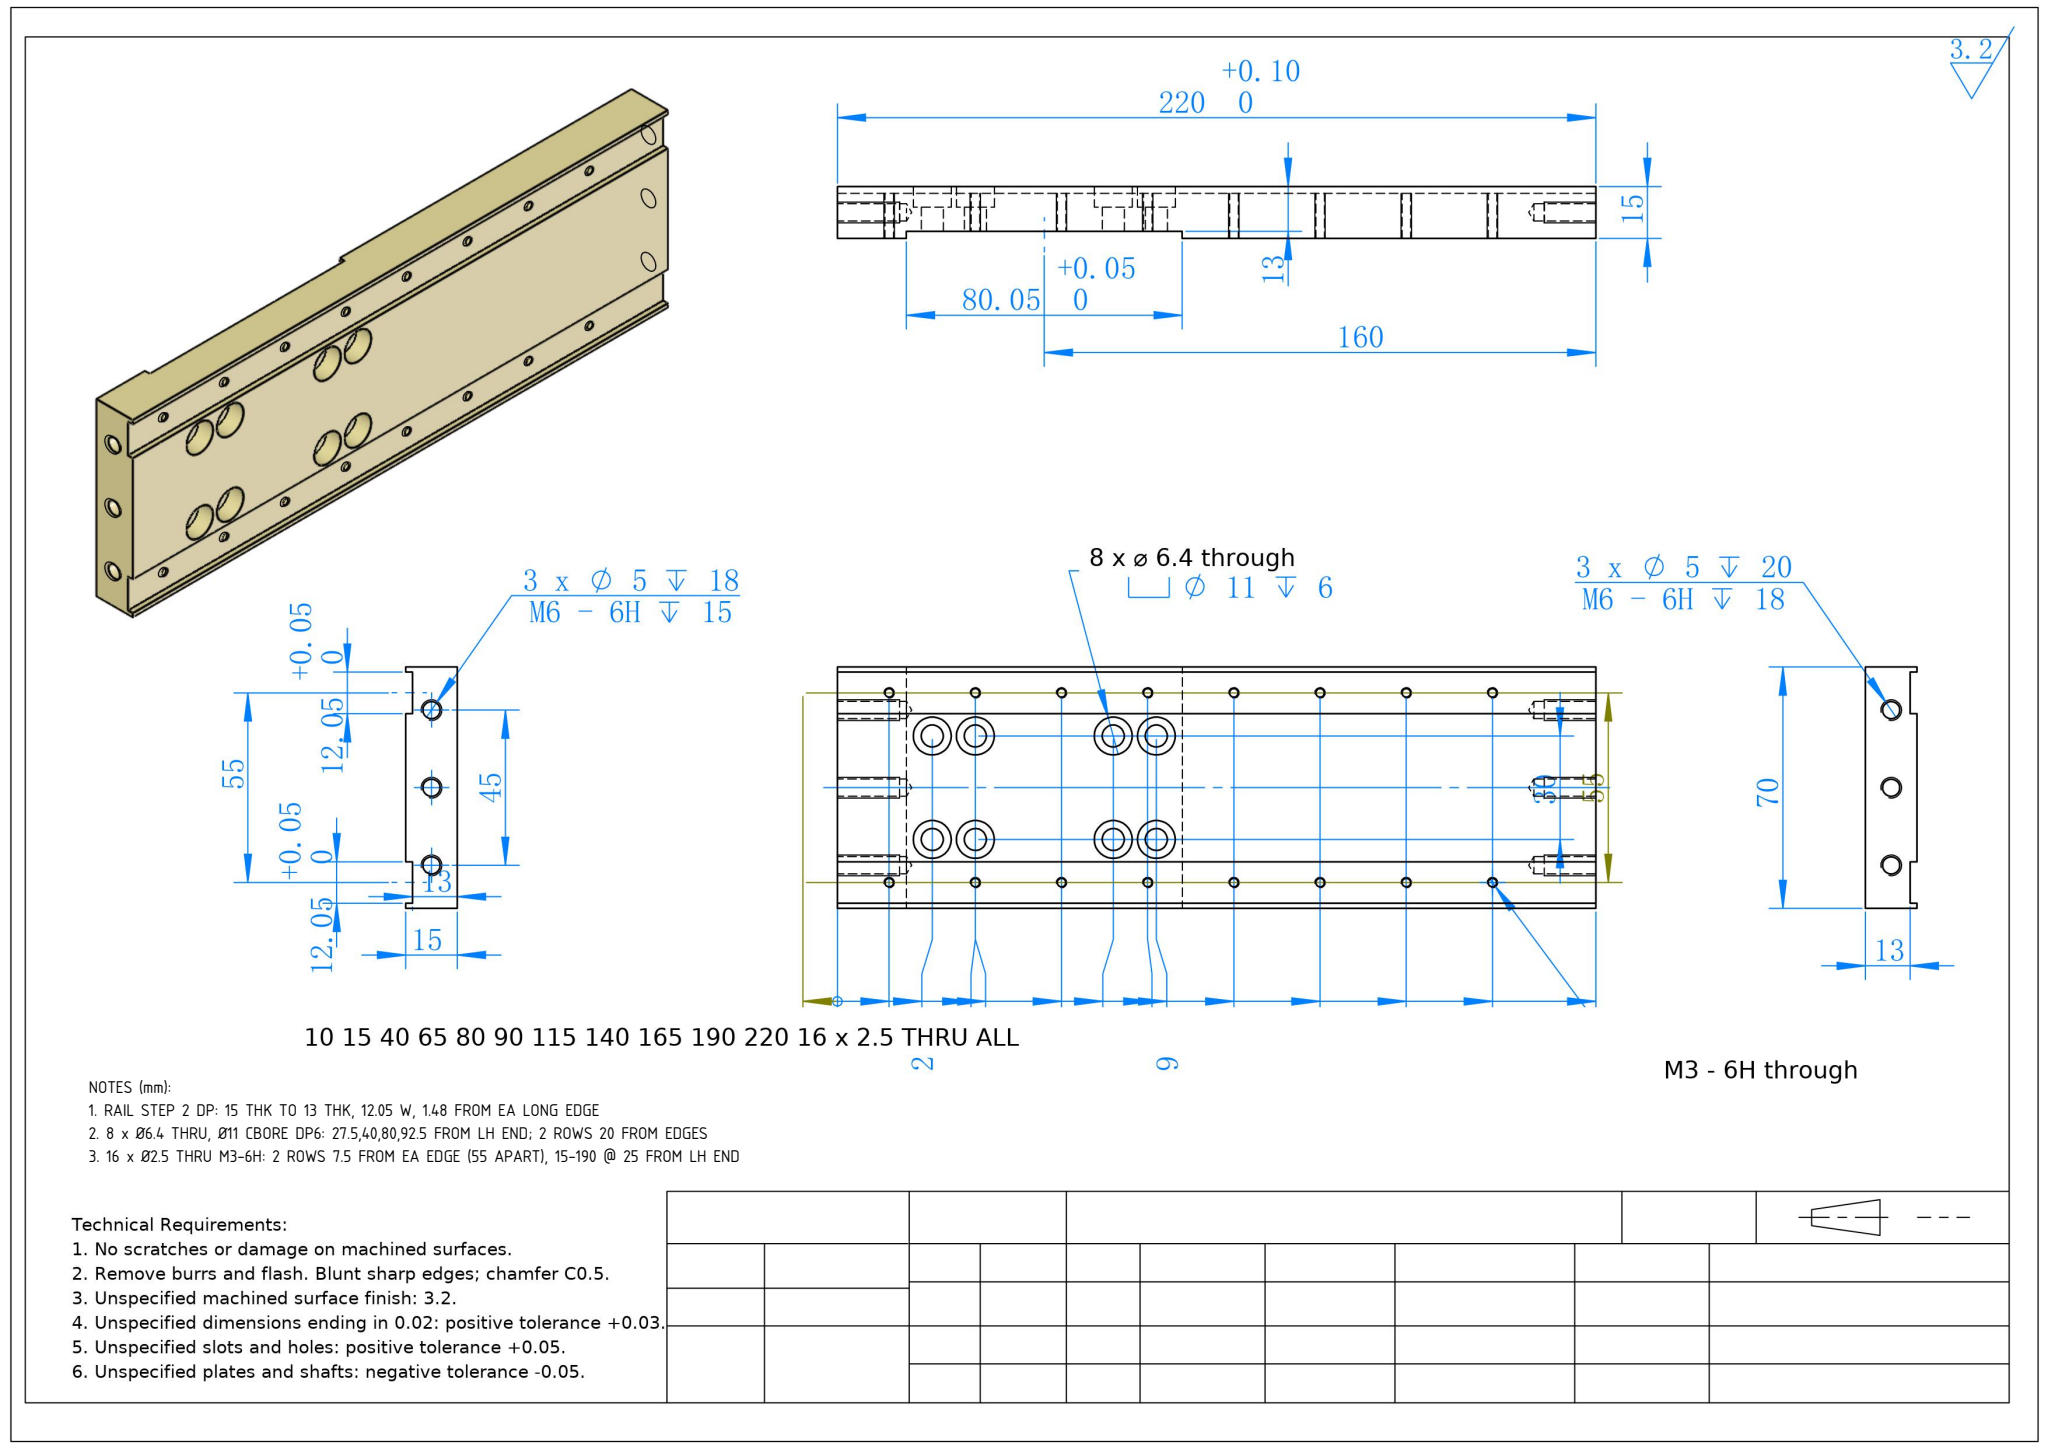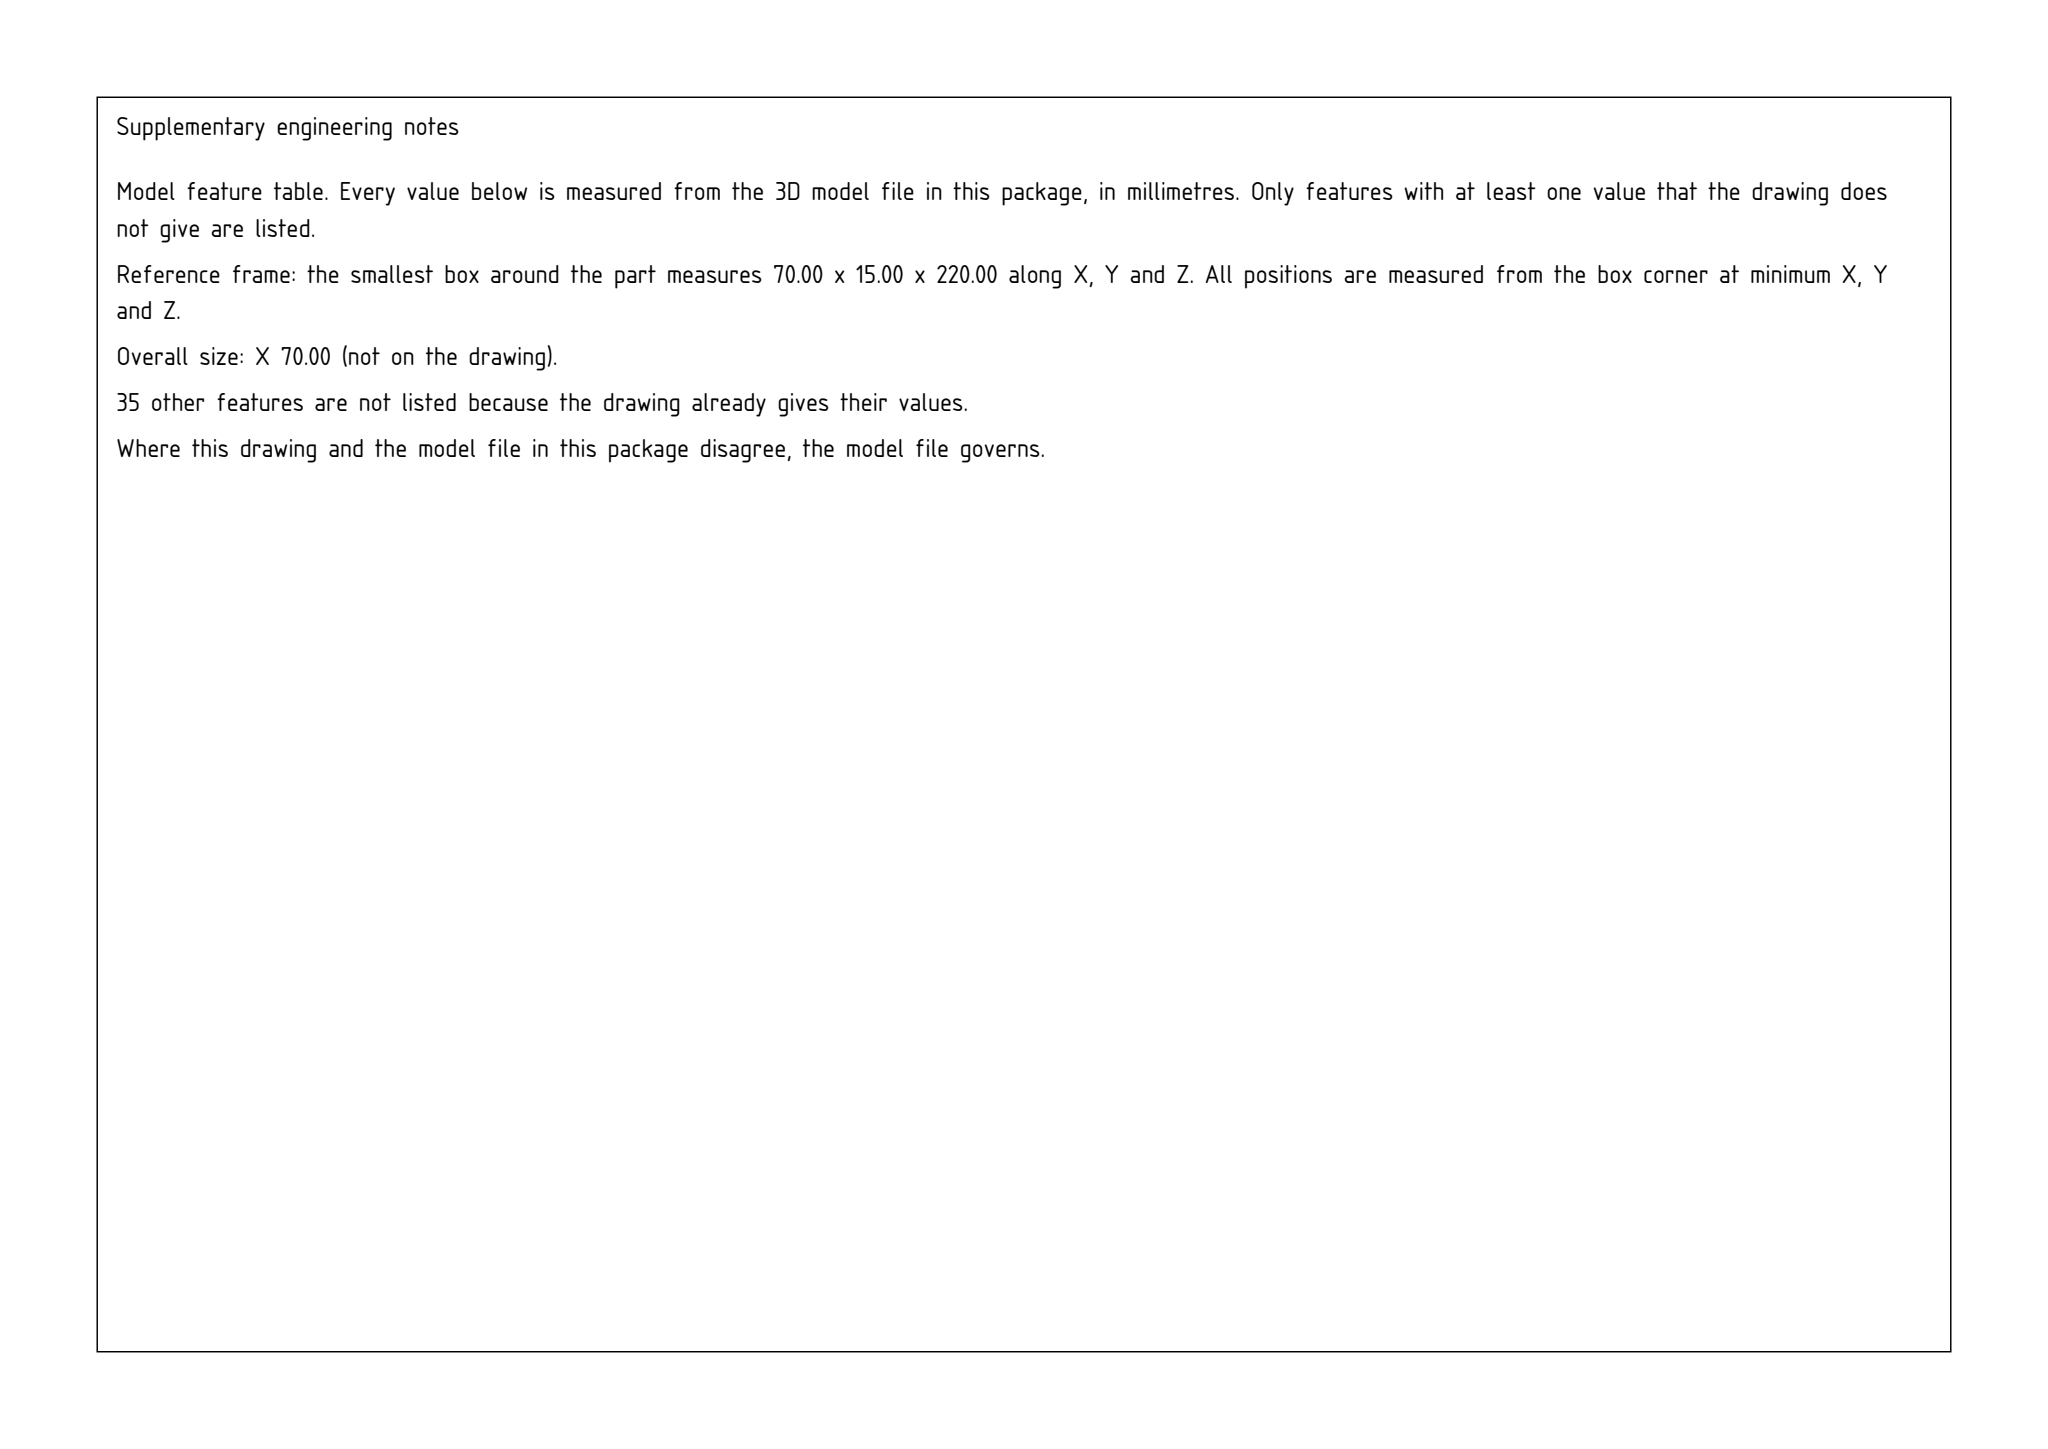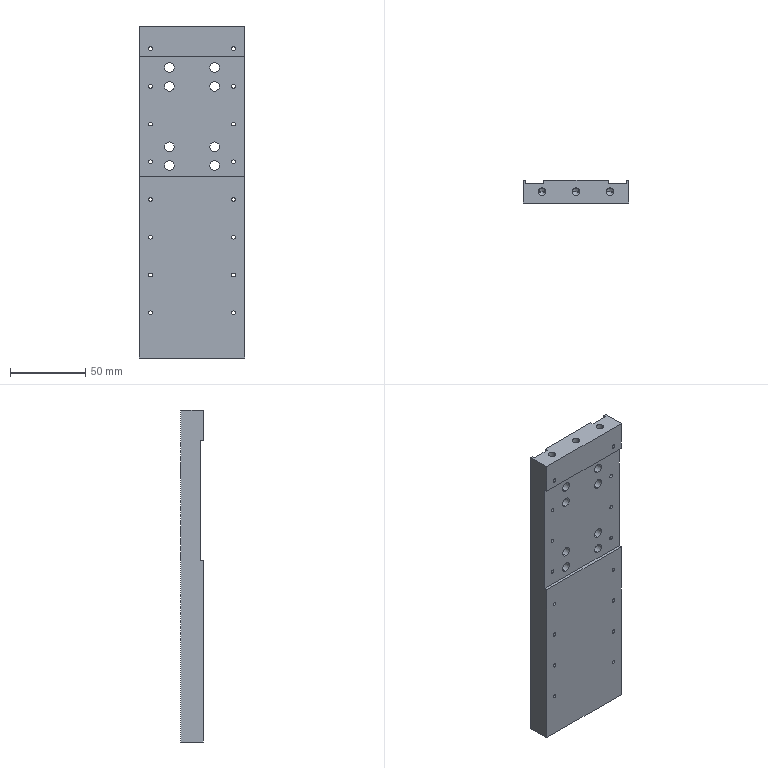Part | SolidWorks | mm | 1 solid | 114 faces | box 70 x 15 x 220 mm | volume 199566 mm3 | cylinder 76 | plane 26 | cone 12 | commonest cylinder face diameters 2.5 x32 11 x16 6.4 x16 5 x12
Drawing notes:
RAIL STEP 2 DP: 15 THK TO 13 THK, 12.05 W, 1.48 FROM EA LONG EDGE | from the solid: y planes 0/2/13/15 = 2 deep step off 15 thk; x planes 1.48,13.53,56.48,68.53 = 12.05 wide, 1.48 in from each edge
8 x Ø6.4 THRU, Ø11 CBORE DP6: 27.5,40,80,92.5 FROM LH END; 2 ROWS 20 FROM EDGES | from the solid: Ø6.4/Ø11 cbore axes along y at x=20 & 50 of 70 wide, z=127.5,140,180,192.5 = 27.5,40,80,92.5 from z=220 LH end; Ø11 ↧6 to y=9
16 x Ø2.5 THRU M3-6H: 2 ROWS 7.5 FROM EA EDGE (55 APART), 15-190 @ 25 FROM LH END | from the solid: Ø2.5 tap-drill axes along y at x=7.5 & 62.5 (55 apart), z=30,55,80,105,130,155,180,205 = 15..190 from LH end, 8 per row
build123d program:
from build123d import *

# Parameters (mm, degrees)
SKETCH1_W                                       = 70
SKETCH1_H                                       = 15
EXTRUDE1_DEPTH                                  = 110
SKETCH16_W                                      = 12.05
SKETCH16_H                                      = 220
CUT_EXTRUDE1_DEPTH                              = 2
SKETCH17_W                                      = 70
SKETCH17_H                                      = 80.05
CUT_EXTRUDE2_DEPTH                              = 2
M6_TAPPED_HOLE3_D                               = 5
M6_TAPPED_HOLE3_DEPTH                           = 18
M6_TAPPED_HOLE3_TIP                             = 1.502
M6_TAPPED_HOLE2_D                               = 5
M6_TAPPED_HOLE2_DEPTH                           = 20
M6_TAPPED_HOLE2_TIP                             = 1.502
M6_HEX_SOCKET_HEAD_CAP_SCREW_CBORE1_D           = 6.4
M6_HEX_SOCKET_HEAD_CAP_SCREW_CBORE1_CBORE_D     = 11
M6_HEX_SOCKET_HEAD_CAP_SCREW_CBORE1_CBORE_DEPTH = 6
M3_TAPPED_HOLE1_D                               = 2.5
LPATTERN1_COUNT                                 = 8
LPATTERN1_PITCH                                 = 25


with BuildPart() as part:
    # Sketch1 → Extrude1 (new, symmetric)
    with BuildSketch(Plane.XY):
        Rectangle(SKETCH1_W, SKETCH1_H)
    extrude(amount=EXTRUDE1_DEPTH, both=True)

    # Sketch16 → Cut-Extrude1 (cut)
    with BuildSketch(Plane(origin=(0, 7.5, 0), x_dir=(1, 0, 0), z_dir=(0, 1, 0))):
        with Locations((27.5, 0)):
            Rectangle(SKETCH16_W, SKETCH16_H)
        with Locations((-27.5, 0)):
            Rectangle(SKETCH16_W, SKETCH16_H)
    extrude(amount=-CUT_EXTRUDE1_DEPTH, mode=Mode.SUBTRACT)

    # Sketch17 → Cut-Extrude2 (cut)
    with BuildSketch(Plane(origin=(0, -7.5, 0), x_dir=(-1, 0, 0), z_dir=(0, -1, 0))):
        with Locations((0, -50)):
            Rectangle(SKETCH17_W, SKETCH17_H)
    extrude(amount=-CUT_EXTRUDE2_DEPTH, mode=Mode.SUBTRACT)

    # M6 Tapped Hole3
    with Locations(Plane(origin=(0, 0, -110), x_dir=(-1, 0, 0), z_dir=(0, 0, -1))):
        with Locations((-22.5, 0), (0, 0), (22.5, 0)):
            Hole(M6_TAPPED_HOLE3_D / 2, depth=M6_TAPPED_HOLE3_DEPTH)
            with Locations((0, 0, -(M6_TAPPED_HOLE3_DEPTH + M6_TAPPED_HOLE3_TIP / 2))):  # 118° drill point
                Cone(0, M6_TAPPED_HOLE3_D / 2, M6_TAPPED_HOLE3_TIP, mode=Mode.SUBTRACT)

    # M6 Tapped Hole2
    with Locations(Plane.XY.offset(110)):
        with Locations((-22.5, 0), (22.5, 0), (0, 0)):
            Hole(M6_TAPPED_HOLE2_D / 2, depth=M6_TAPPED_HOLE2_DEPTH)
            with Locations((0, 0, -(M6_TAPPED_HOLE2_DEPTH + M6_TAPPED_HOLE2_TIP / 2))):  # 118° drill point
                Cone(0, M6_TAPPED_HOLE2_D / 2, M6_TAPPED_HOLE2_TIP, mode=Mode.SUBTRACT)

    # M6 Hex Socket Head Cap Screw CBORE1 (through all)
    with Locations(Plane(origin=(0, 7.5, 0), x_dir=(1, 0, 0), z_dir=(0, 1, 0))):
        with Locations((15, -30), (-15, -30), (15, -70), (-15, -70), (-15, -82.5), (15, -82.5), (-15, -17.5), (15, -17.5)):
            CounterBoreHole(M6_HEX_SOCKET_HEAD_CAP_SCREW_CBORE1_D / 2, M6_HEX_SOCKET_HEAD_CAP_SCREW_CBORE1_CBORE_D / 2, M6_HEX_SOCKET_HEAD_CAP_SCREW_CBORE1_CBORE_DEPTH)

    # M3 Tapped Hole1 (through all)
    with Locations(Plane(origin=(0, 7.5, 0), x_dir=(-1, 0, 0), z_dir=(0, 1, 0))):
        with Locations((-27.5, -80), (27.5, -80)):
            m3_tapped_hole1 = Hole(M3_TAPPED_HOLE1_D / 2)

    # LPattern1: M3 Tapped Hole1 ×8
    with Locations(*[(0, 0, i * LPATTERN1_PITCH) for i in range(1, LPATTERN1_COUNT)]):
        add(m3_tapped_hole1, mode=Mode.SUBTRACT)


solid = part.part